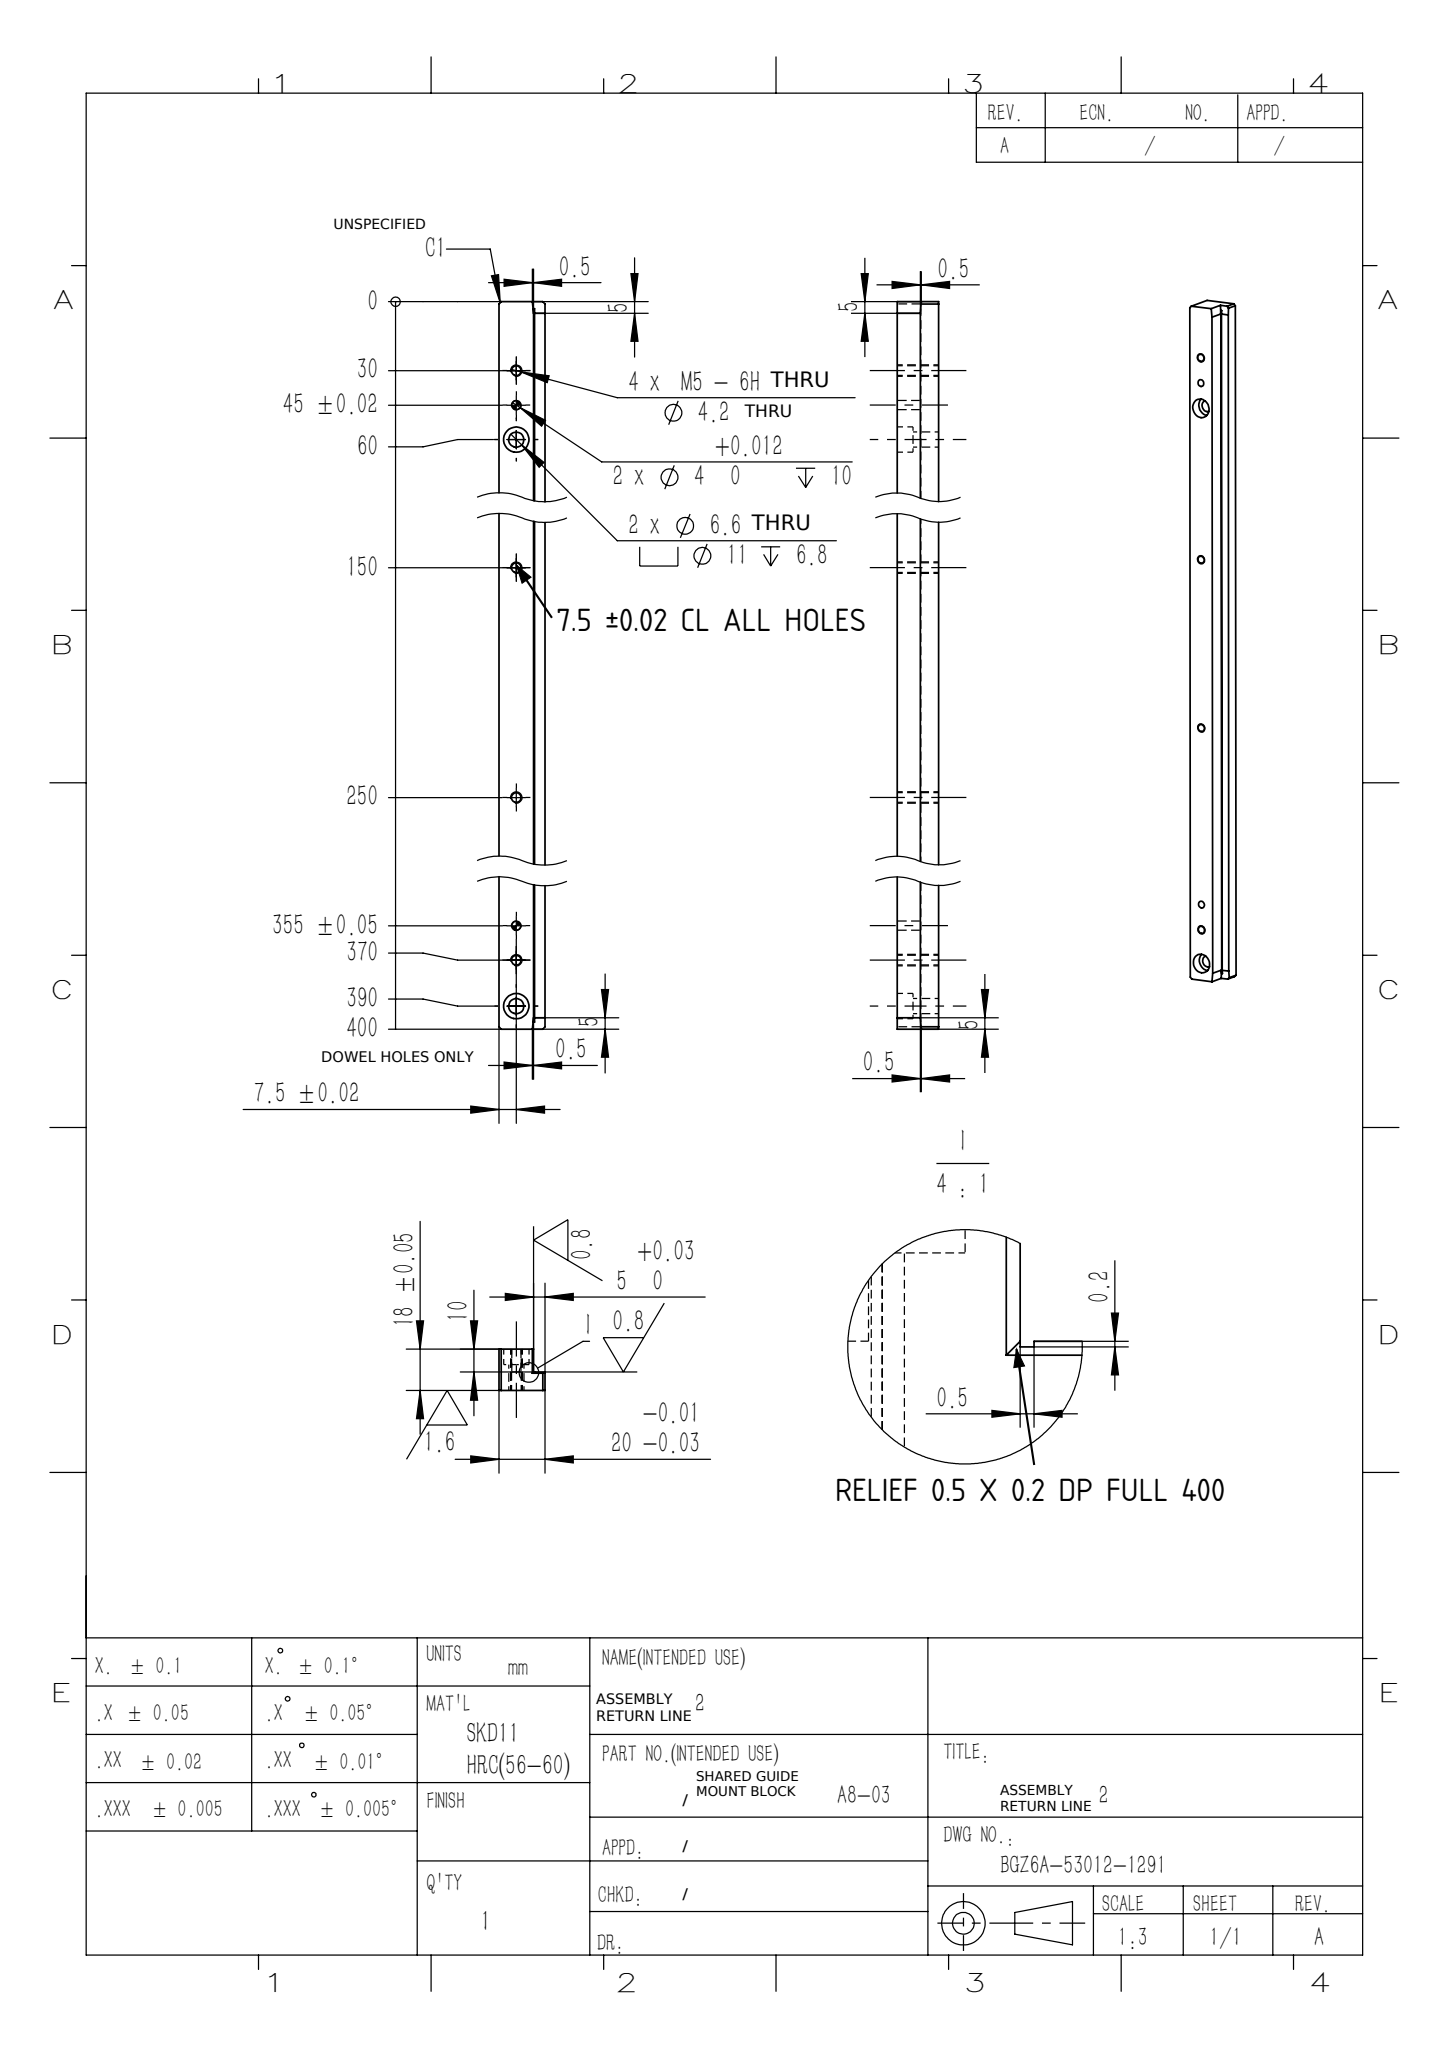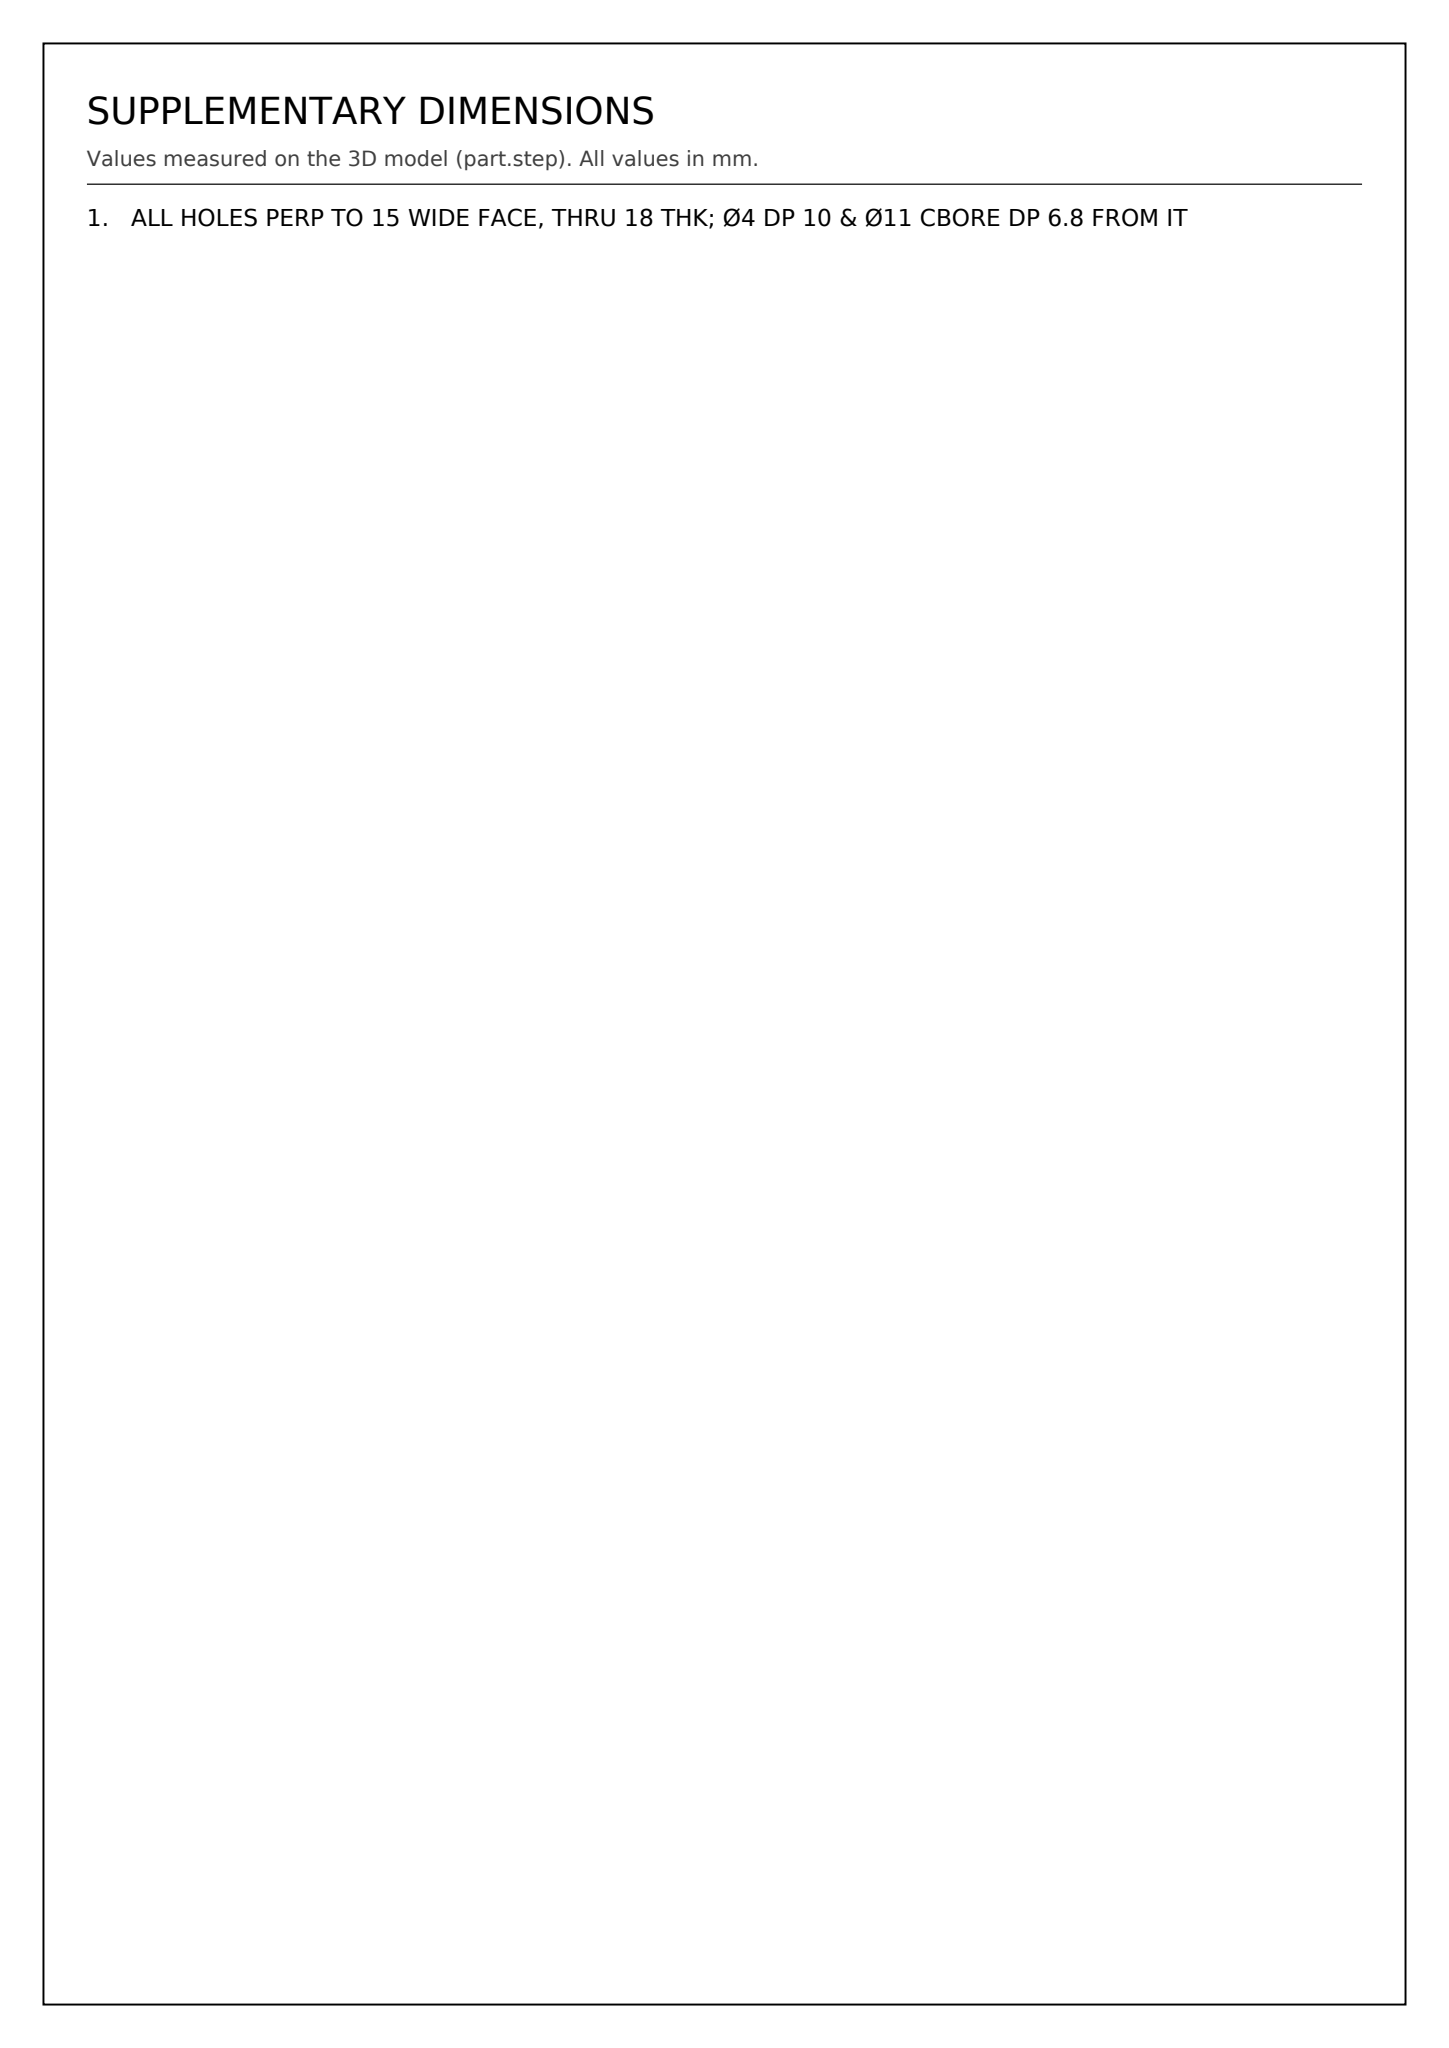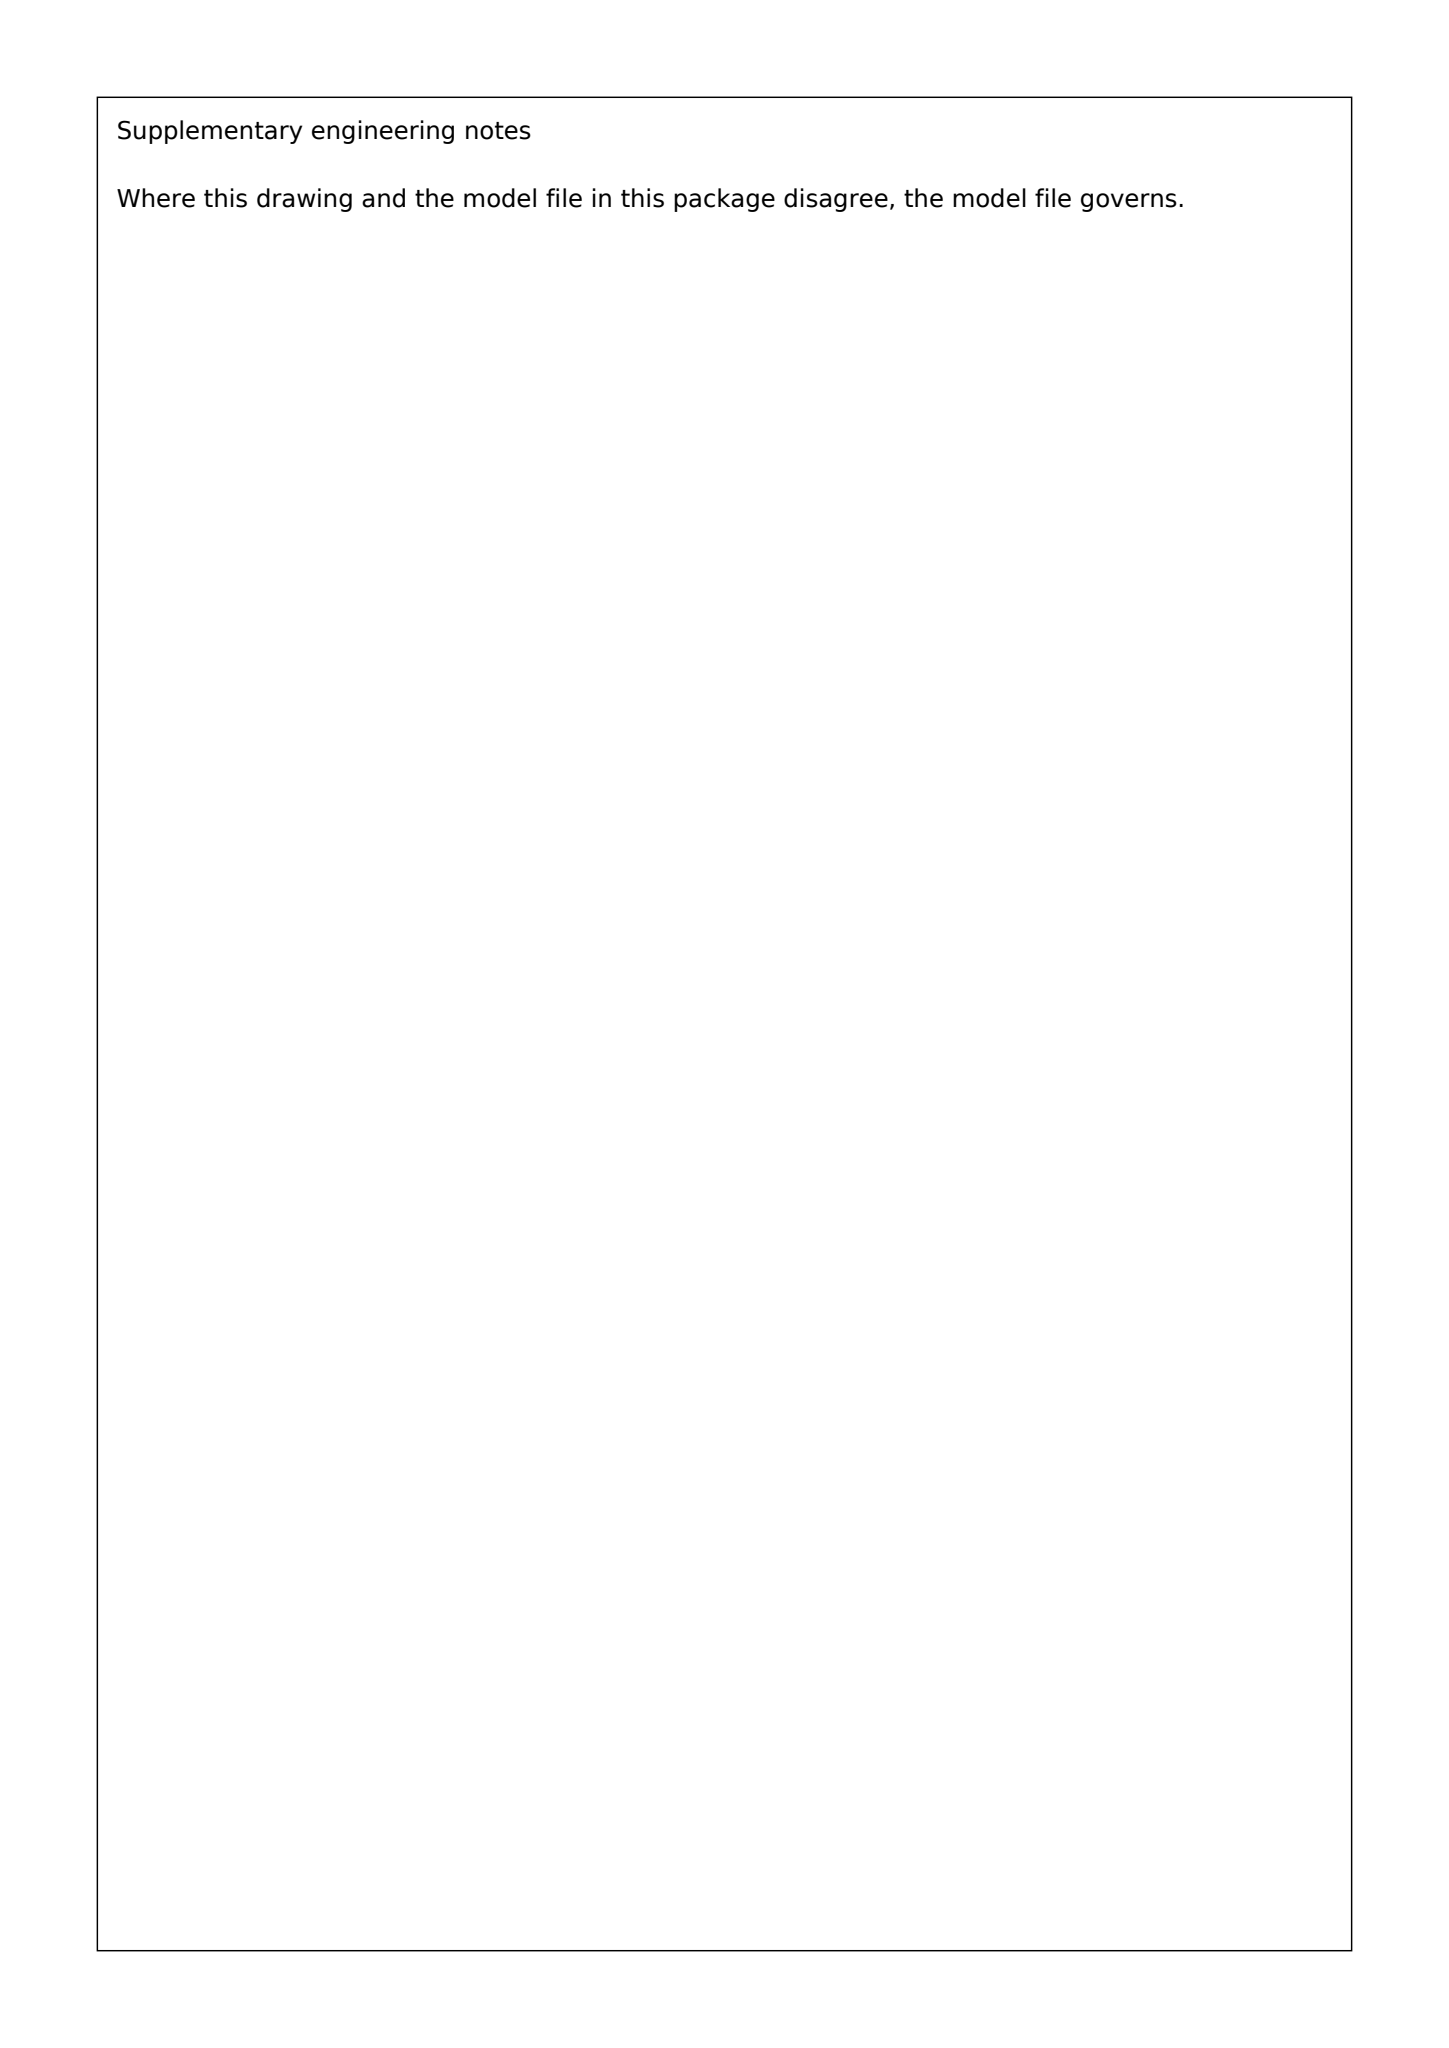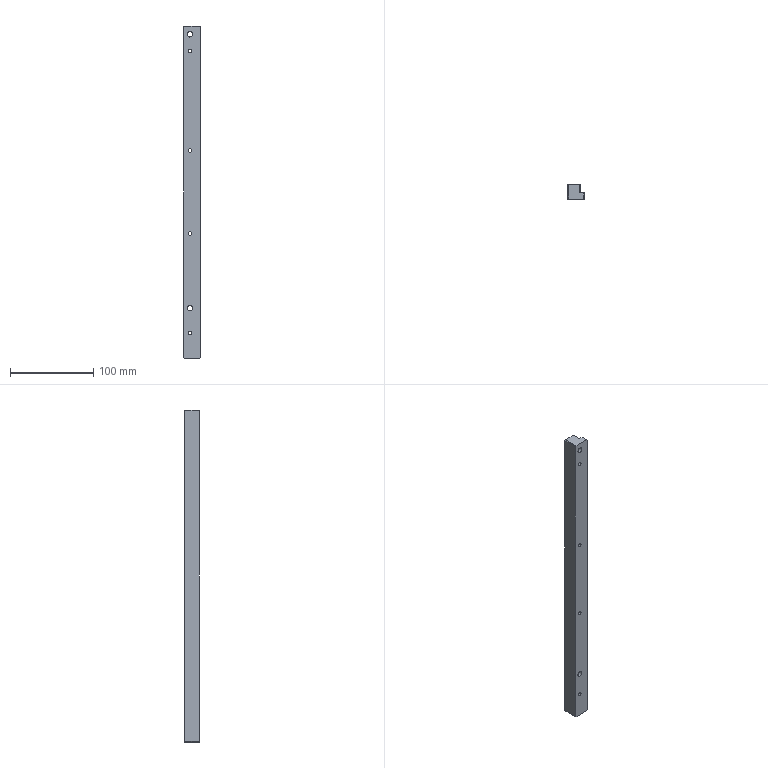Part | SolidWorks | mm | material SKD11 | 1 solid | 42 faces | box 20 x 18 x 400 mm | volume 120589 mm3 | plane 22 | cylinder 20 | commonest cylinder face diameters 4.2 x8 11 x4 6.6 x4 4 x4
Drawing notes:
7.5 ±0.02 CL APPLIES TO ALL HOLES, NOT DOWEL HOLES ONLY | from the solid: All cylinders (Ø4, Ø4.2, Ø6.6, Ø11) at x = 7.5 in 20 wide bbox
ALL HOLES PERP TO 15 WIDE FACE, THRU 18 THK; Ø4 DP 10 & Ø11 CBORE DP 6.8 FROM IT | from the solid: Cyl axes = y, thk y=18; Ø4 L10 ends y=8.0; Ø11 L6.8 ends y=11.2; Ø6.6 L11.2 from y=0
CORNER RELIEF 0.5 X 0.2 DP FULL 400 LG, THRU BOTH ENDS | from the solid: x planes 15/15.5 and y planes 7.8/8.0; only z planes are 0 and 400
build123d program:
from build123d import *
from OCP.BRepFilletAPI import BRepFilletAPI_MakeChamfer

# Parameters (mm, degrees)
BOSS_EXTRUDE1_DEPTH                             = 400
CHAMFER1_SIZE                                   = 0.5
CHAMFER1_SIZE2                                  = 5.001
SKETCH2_W                                       = 0.5
SKETCH2_H                                       = 0.2
CUT_EXTRUDE1_DEPTH                              = 401.904
CHAMFER2_SIZE                                   = 1
F_4_0MM_DOWEL_PIN_HOLE_2_D                      = 4
F_4_0MM_DOWEL_PIN_HOLE_2_DEPTH                  = 10
M5_TAPPED_HOLE2_D                               = 4.2
M6_HEX_SOCKET_HEAD_CAP_SCREW_CBORE1_D           = 6.6
M6_HEX_SOCKET_HEAD_CAP_SCREW_CBORE1_CBORE_D     = 11
M6_HEX_SOCKET_HEAD_CAP_SCREW_CBORE1_CBORE_DEPTH = 6.8


with BuildPart() as part:
    # Sketch1 → Boss-Extrude1 (new body)
    with BuildSketch(Plane.XY):
        Polygon((0, 0), (0, 18), (15, 18), (15, 8), (20, 8), (20, 0), align=None)
    extrude(amount=BOSS_EXTRUDE1_DEPTH)

    # Chamfer1: one chamfer whose edges measure the first distance from different faces: ONE call of the kernel's chamfer builder (chamfer() names one face for all edges)
    chamfer1_edges_1 = [part.edges().sort_by_distance(p)[0] for p in [
        (17.5, 8, 400),
        (15, 13, 400),
    ]]
    chamfer1_side_1 = [part.faces().sort_by_distance(p)[0] for p in [
        (8.79, 8.355, 400),
    ]]
    chamfer1_edges_2 = [part.edges().sort_by_distance(p)[0] for p in [
        (15, 13, 0),
        (17.5, 8, 0),
    ]]
    chamfer1_side_2 = [part.faces().sort_by_distance(p)[0] for p in [
        (8.79, 8.355, 0),
    ]]
    chamfer1 = BRepFilletAPI_MakeChamfer(part.part.solid().wrapped)
    for e in chamfer1_edges_1:
        chamfer1.Add(CHAMFER1_SIZE, CHAMFER1_SIZE2, e.wrapped, chamfer1_side_1[0].wrapped)  # the first distance lies on this face
    for e in chamfer1_edges_2:
        chamfer1.Add(CHAMFER1_SIZE, CHAMFER1_SIZE2, e.wrapped, chamfer1_side_2[0].wrapped)  # the first distance lies on this face
    add(Compound.cast(chamfer1.Shape()), mode=Mode.REPLACE)

    # Sketch2 → Cut-Extrude1 (cut, through all)
    with BuildSketch(Plane.XY.offset(400)):
        with Locations((15.25, 7.9)):
            Rectangle(SKETCH2_W, SKETCH2_H)
    extrude(amount=-CUT_EXTRUDE1_DEPTH, mode=Mode.SUBTRACT)

    # Chamfer2
    chamfer2_edges = [part.edges().sort_by_distance(p)[0] for p in [
        (0, 9, 400),
        (0, 9, 0),
        (20, 3.75, 0),
        (20, 3.75, 400),
    ]]
    chamfer(chamfer2_edges, length=CHAMFER2_SIZE)

    # 4.0mm Dowel Pin Hole 2
    with Locations(Plane(origin=(0, 18, 0), x_dir=(1, 0, 0), z_dir=(0, 1, 0))):
        with Locations((7.5, -45), (7.5, -355)):
            Hole(F_4_0MM_DOWEL_PIN_HOLE_2_D / 2, depth=F_4_0MM_DOWEL_PIN_HOLE_2_DEPTH)

    # M5 Tapped Hole2 (through all)
    with Locations(Plane(origin=(0, 18, 0), x_dir=(1, 0, 0), z_dir=(0, 1, 0))):
        with Locations((7.5, -370), (7.5, -150), (7.5, -30), (7.5, -250)):
            Hole(M5_TAPPED_HOLE2_D / 2)

    # M6 Hex Socket Head Cap Screw CBORE1 (through all)
    with Locations(Plane(origin=(0, 18, 0), x_dir=(1, 0, 0), z_dir=(0, 1, 0))):
        with Locations((7.5, -390), (7.5, -60)):
            CounterBoreHole(M6_HEX_SOCKET_HEAD_CAP_SCREW_CBORE1_D / 2, M6_HEX_SOCKET_HEAD_CAP_SCREW_CBORE1_CBORE_D / 2, M6_HEX_SOCKET_HEAD_CAP_SCREW_CBORE1_CBORE_DEPTH)


solid = part.part